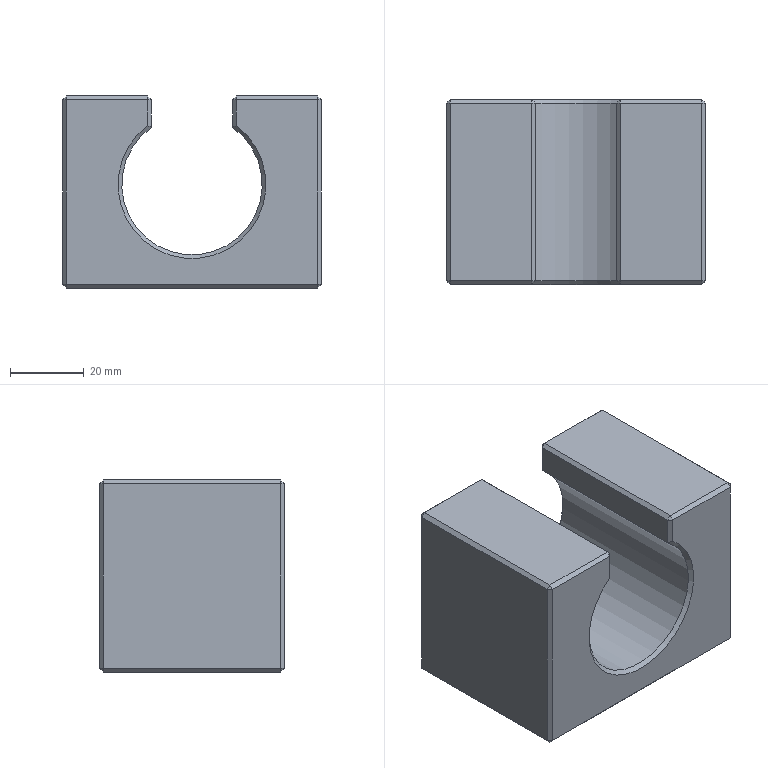CAM job | Mastercam | mm | 9 operations | part box 70 x 50 x 52
1. Facing | 20 - 63 平铣刀
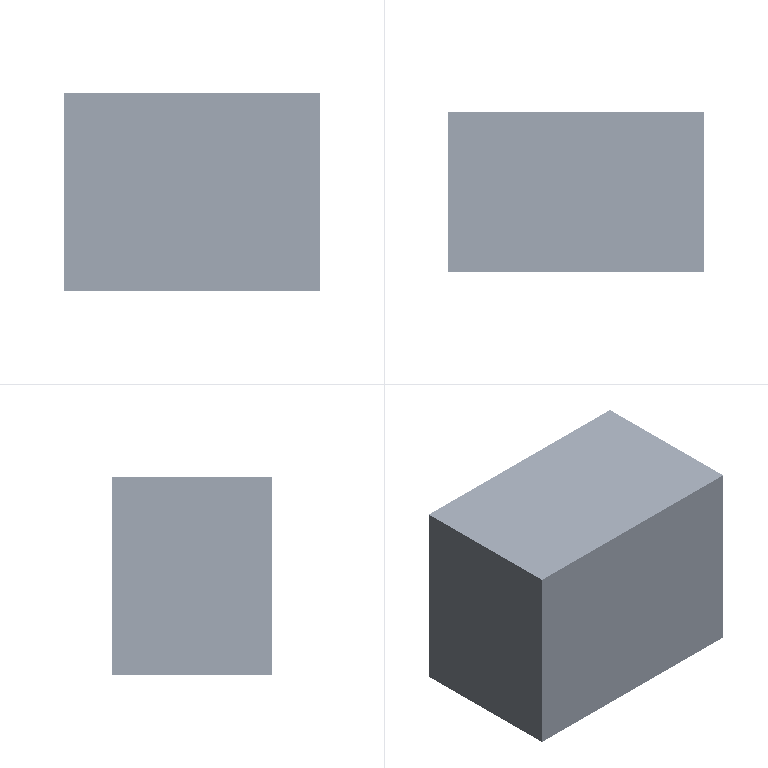2. 2D High Speed (2D Dynamic Mill) | 16 - 16 平铣刀
3. Contour (2D) | 16 - 16 平铣刀
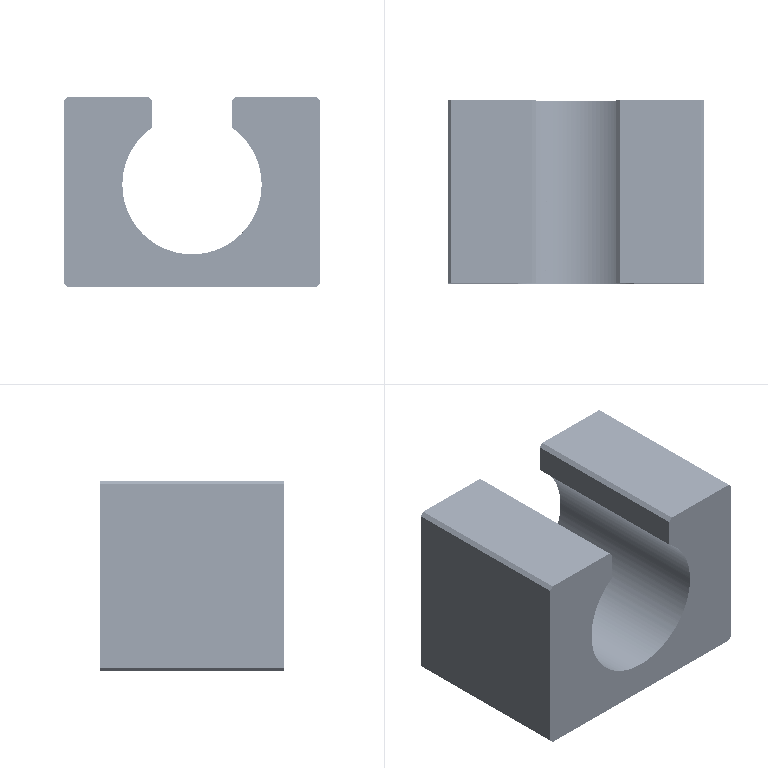4. Contour (2D) | 16 - 16 平铣刀
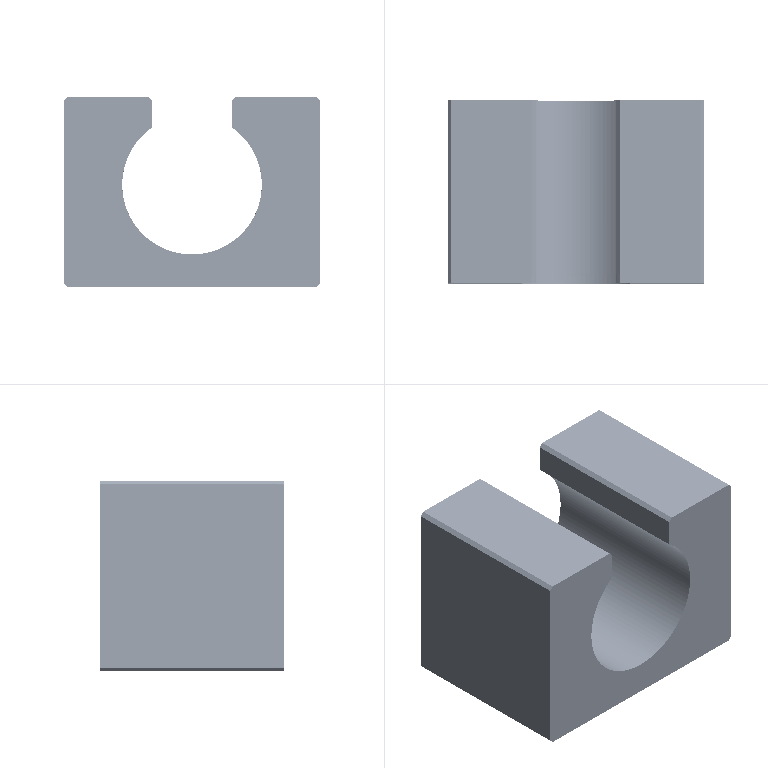5. Drill/Counterbore | 7 - 4 倒角刀
6. Contour (2D chamfer) | 7 - 4 倒角刀
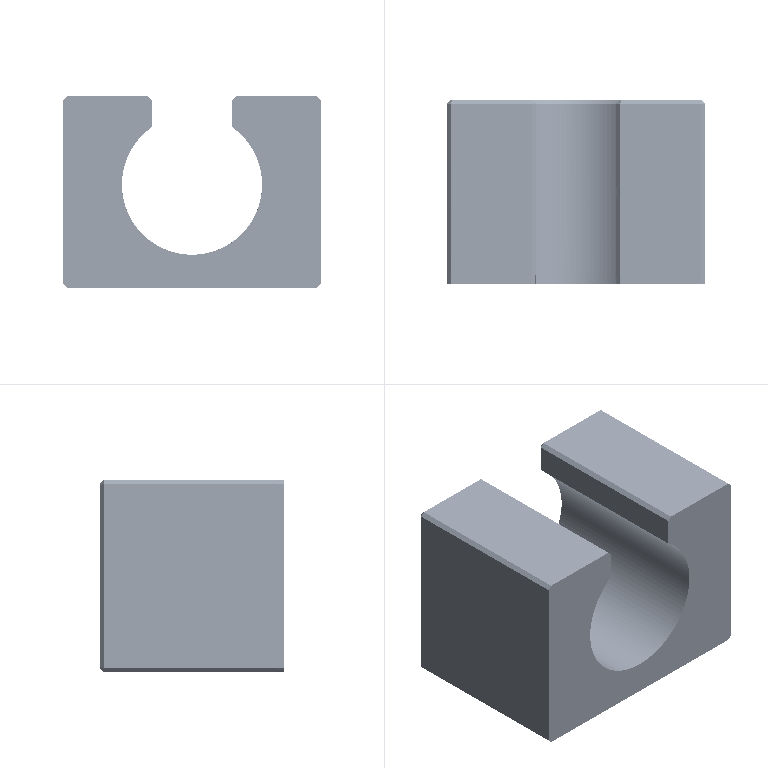7. Facing | 20 - 63 平铣刀
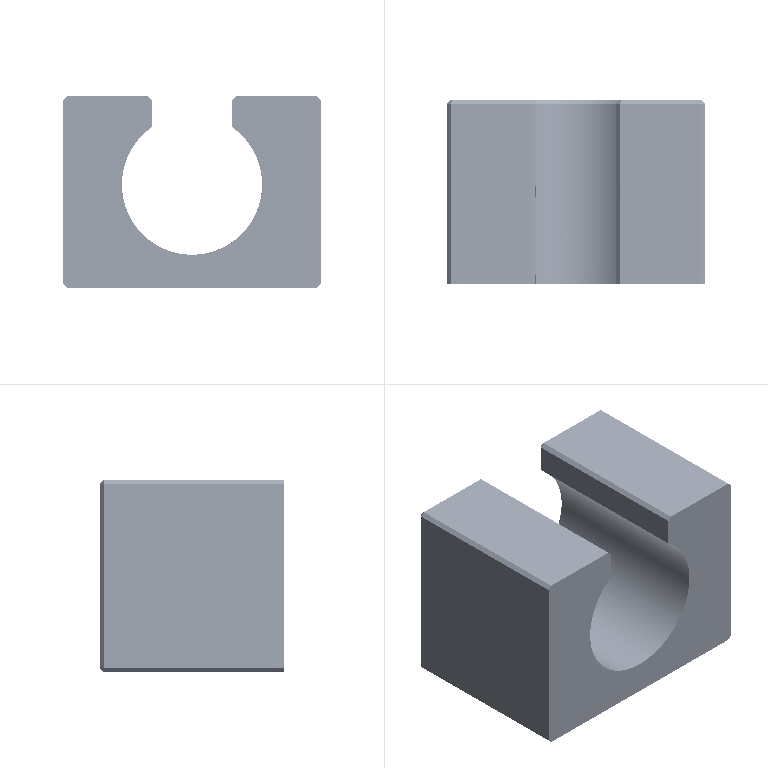8. Contour (2D chamfer) | 7 - 4 倒角刀
9. Drill/Counterbore | 7 - 4 倒角刀